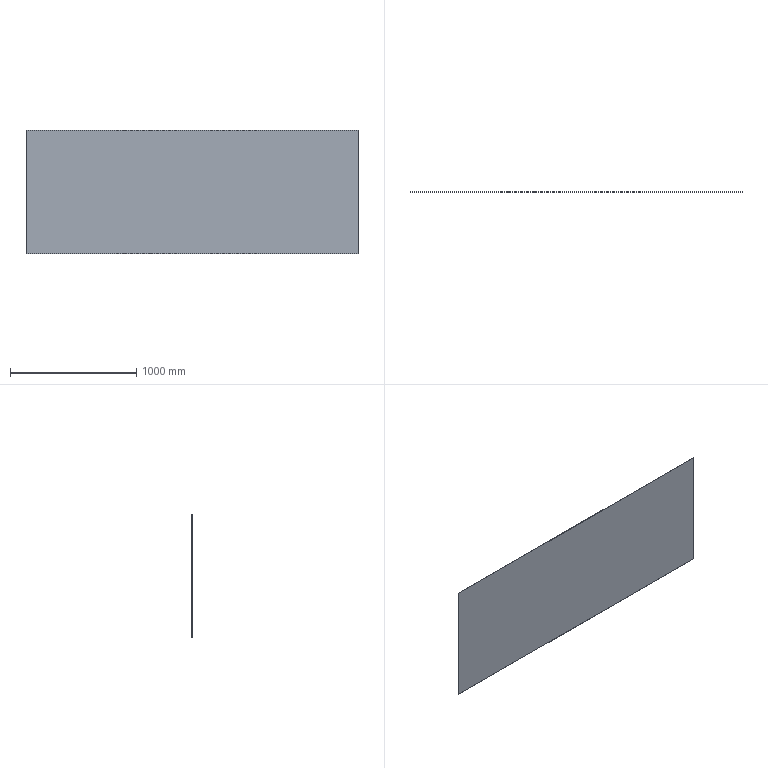Component | NX | TOP_COVER | 1 solid | 6 faces | box 2630 x 2 x 980 mm | volume 5154800 mm3 | plane 6
STEP:
#1=CARTESIAN_POINT('',(0.,0.,0.));
#2=DIRECTION('',(0.,0.,1.));
#3=DIRECTION('',(1.,0.,0.));
#4=AXIS2_PLACEMENT_3D('',#1,#2,#3);
#5=CARTESIAN_POINT('',(1972.985,1609.529,-1766.475));
#6=VERTEX_POINT('',#5);
#7=CARTESIAN_POINT('',(-657.015,1609.529,-1766.475));
#8=VERTEX_POINT('',#7);
#9=CARTESIAN_POINT('',(1972.985,1609.529,-1766.475));
#10=DIRECTION('',(-1.,0.,-0.));
#11=VECTOR('',#10,1.);
#12=LINE('',#9,#11);
#13=CARTESIAN_POINT('',(1972.985,1611.529,-1766.475));
#14=DIRECTION('',(-0.,0.,1.));
#15=DIRECTION('',(-1.,0.,-0.));
#16=AXIS2_PLACEMENT_3D('',#13,#14,#15);
#17=PLANE('',#16);
#18=CARTESIAN_POINT('',(0.,2.));
#19=DIRECTION('',(1.,0.));
#20=VECTOR('',#19,1.);
#21=LINE('',#18,#20);
#22=(GEOMETRIC_REPRESENTATION_CONTEXT(2)PARAMETRIC_REPRESENTATION_CONTEXT()REPRESENTATION_CONTEXT('',''));
#23=DEFINITIONAL_REPRESENTATION('',(#21),#22);
#24=PCURVE('',#17,#23);
#25=CARTESIAN_POINT('',(-657.015,1609.529,-2746.475));
#26=DIRECTION('',(0.,-1.,0.));
#27=DIRECTION('',(1.,0.,0.));
#28=AXIS2_PLACEMENT_3D('',#25,#26,#27);
#29=PLANE('',#28);
#30=CARTESIAN_POINT('',(2630.,980.));
#31=DIRECTION('',(-1.,-0.));
#32=VECTOR('',#31,1.);
#33=LINE('',#30,#32);
#34=(GEOMETRIC_REPRESENTATION_CONTEXT(2)PARAMETRIC_REPRESENTATION_CONTEXT()REPRESENTATION_CONTEXT('',''));
#35=DEFINITIONAL_REPRESENTATION('',(#33),#34);
#36=PCURVE('',#29,#35);
#37=SURFACE_CURVE('',#12,(#24,#36),.PCURVE_S1.);
#38=EDGE_CURVE('',#6,#8,#37,.T.);
#39=ORIENTED_EDGE('',*,*,#38,.F.);
#40=CARTESIAN_POINT('',(1972.985,1611.529,-1766.475));
#41=VERTEX_POINT('',#40);
#42=CARTESIAN_POINT('',(1972.985,1611.529,-1766.475));
#43=DIRECTION('',(0.,-1.,0.));
#44=VECTOR('',#43,1.);
#45=LINE('',#42,#44);
#46=CARTESIAN_POINT('',(0.,0.));
#47=DIRECTION('',(0.,1.));
#48=VECTOR('',#47,1.);
#49=LINE('',#46,#48);
#50=(GEOMETRIC_REPRESENTATION_CONTEXT(2)PARAMETRIC_REPRESENTATION_CONTEXT()REPRESENTATION_CONTEXT('',''));
#51=DEFINITIONAL_REPRESENTATION('',(#49),#50);
#52=PCURVE('',#17,#51);
#53=CARTESIAN_POINT('',(1972.985,1611.529,-2746.475));
#54=DIRECTION('',(1.,0.,0.));
#55=DIRECTION('',(0.,1.,0.));
#56=AXIS2_PLACEMENT_3D('',#53,#54,#55);
#57=PLANE('',#56);
#58=CARTESIAN_POINT('',(0.,980.));
#59=DIRECTION('',(-1.,0.));
#60=VECTOR('',#59,1.);
#61=LINE('',#58,#60);
#62=(GEOMETRIC_REPRESENTATION_CONTEXT(2)PARAMETRIC_REPRESENTATION_CONTEXT()REPRESENTATION_CONTEXT('',''));
#63=DEFINITIONAL_REPRESENTATION('',(#61),#62);
#64=PCURVE('',#57,#63);
#65=SURFACE_CURVE('',#45,(#52,#64),.PCURVE_S1.);
#66=EDGE_CURVE('',#41,#6,#65,.T.);
#67=ORIENTED_EDGE('',*,*,#66,.F.);
#68=CARTESIAN_POINT('',(-657.015,1611.529,-1766.475));
#69=VERTEX_POINT('',#68);
#70=CARTESIAN_POINT('',(1972.985,1611.529,-1766.475));
#71=DIRECTION('',(-1.,0.,-0.));
#72=VECTOR('',#71,1.);
#73=LINE('',#70,#72);
#74=CARTESIAN_POINT('',(0.,0.));
#75=DIRECTION('',(1.,0.));
#76=VECTOR('',#75,1.);
#77=LINE('',#74,#76);
#78=(GEOMETRIC_REPRESENTATION_CONTEXT(2)PARAMETRIC_REPRESENTATION_CONTEXT()REPRESENTATION_CONTEXT('',''));
#79=DEFINITIONAL_REPRESENTATION('',(#77),#78);
#80=PCURVE('',#17,#79);
#81=CARTESIAN_POINT('',(-657.015,1611.529,-2746.475));
#82=DIRECTION('',(0.,-1.,0.));
#83=DIRECTION('',(1.,0.,0.));
#84=AXIS2_PLACEMENT_3D('',#81,#82,#83);
#85=PLANE('',#84);
#86=CARTESIAN_POINT('',(2630.,980.));
#87=DIRECTION('',(-1.,-0.));
#88=VECTOR('',#87,1.);
#89=LINE('',#86,#88);
#90=(GEOMETRIC_REPRESENTATION_CONTEXT(2)PARAMETRIC_REPRESENTATION_CONTEXT()REPRESENTATION_CONTEXT('',''));
#91=DEFINITIONAL_REPRESENTATION('',(#89),#90);
#92=PCURVE('',#85,#91);
#93=SURFACE_CURVE('',#73,(#80,#92),.PCURVE_S1.);
#94=EDGE_CURVE('',#41,#69,#93,.T.);
#95=ORIENTED_EDGE('',*,*,#94,.T.);
#96=CARTESIAN_POINT('',(-657.015,1611.529,-1766.475));
#97=DIRECTION('',(0.,-1.,0.));
#98=VECTOR('',#97,1.);
#99=LINE('',#96,#98);
#100=CARTESIAN_POINT('',(2630.,0.));
#101=DIRECTION('',(0.,1.));
#102=VECTOR('',#101,1.);
#103=LINE('',#100,#102);
#104=(GEOMETRIC_REPRESENTATION_CONTEXT(2)PARAMETRIC_REPRESENTATION_CONTEXT()REPRESENTATION_CONTEXT('',''));
#105=DEFINITIONAL_REPRESENTATION('',(#103),#104);
#106=PCURVE('',#17,#105);
#107=CARTESIAN_POINT('',(-657.015,1611.529,-1766.475));
#108=DIRECTION('',(-1.,0.,0.));
#109=DIRECTION('',(0.,-1.,0.));
#110=AXIS2_PLACEMENT_3D('',#107,#108,#109);
#111=PLANE('',#110);
#112=CARTESIAN_POINT('',(0.,0.));
#113=DIRECTION('',(1.,0.));
#114=VECTOR('',#113,1.);
#115=LINE('',#112,#114);
#116=(GEOMETRIC_REPRESENTATION_CONTEXT(2)PARAMETRIC_REPRESENTATION_CONTEXT()REPRESENTATION_CONTEXT('',''));
#117=DEFINITIONAL_REPRESENTATION('',(#115),#116);
#118=PCURVE('',#111,#117);
#119=SURFACE_CURVE('',#99,(#106,#118),.PCURVE_S1.);
#120=EDGE_CURVE('',#69,#8,#119,.T.);
#121=ORIENTED_EDGE('',*,*,#120,.T.);
#122=EDGE_LOOP('',(#39,#67,#95,#121));
#123=FACE_BOUND('',#122,.T.);
#124=ADVANCED_FACE('',(#123),#17,.T.);
#125=CARTESIAN_POINT('',(-657.015,1609.529,-2746.475));
#126=VERTEX_POINT('',#125);
#127=CARTESIAN_POINT('',(-657.015,1609.529,-1766.475));
#128=DIRECTION('',(0.,0.,-1.));
#129=VECTOR('',#128,1.);
#130=LINE('',#127,#129);
#131=CARTESIAN_POINT('',(2.,0.));
#132=DIRECTION('',(0.,-1.));
#133=VECTOR('',#132,1.);
#134=LINE('',#131,#133);
#135=(GEOMETRIC_REPRESENTATION_CONTEXT(2)PARAMETRIC_REPRESENTATION_CONTEXT()REPRESENTATION_CONTEXT('',''));
#136=DEFINITIONAL_REPRESENTATION('',(#134),#135);
#137=PCURVE('',#111,#136);
#138=CARTESIAN_POINT('',(0.,980.));
#139=DIRECTION('',(0.,-1.));
#140=VECTOR('',#139,1.);
#141=LINE('',#138,#140);
#142=(GEOMETRIC_REPRESENTATION_CONTEXT(2)PARAMETRIC_REPRESENTATION_CONTEXT()REPRESENTATION_CONTEXT('',''));
#143=DEFINITIONAL_REPRESENTATION('',(#141),#142);
#144=PCURVE('',#29,#143);
#145=SURFACE_CURVE('',#130,(#137,#144),.PCURVE_S1.);
#146=EDGE_CURVE('',#8,#126,#145,.T.);
#147=ORIENTED_EDGE('',*,*,#146,.F.);
#148=ORIENTED_EDGE('',*,*,#120,.F.);
#149=CARTESIAN_POINT('',(-657.015,1611.529,-2746.475));
#150=VERTEX_POINT('',#149);
#151=CARTESIAN_POINT('',(-657.015,1611.529,-1766.475));
#152=DIRECTION('',(0.,0.,-1.));
#153=VECTOR('',#152,1.);
#154=LINE('',#151,#153);
#155=CARTESIAN_POINT('',(0.,0.));
#156=DIRECTION('',(0.,-1.));
#157=VECTOR('',#156,1.);
#158=LINE('',#155,#157);
#159=(GEOMETRIC_REPRESENTATION_CONTEXT(2)PARAMETRIC_REPRESENTATION_CONTEXT()REPRESENTATION_CONTEXT('',''));
#160=DEFINITIONAL_REPRESENTATION('',(#158),#159);
#161=PCURVE('',#111,#160);
#162=CARTESIAN_POINT('',(0.,980.));
#163=DIRECTION('',(0.,-1.));
#164=VECTOR('',#163,1.);
#165=LINE('',#162,#164);
#166=(GEOMETRIC_REPRESENTATION_CONTEXT(2)PARAMETRIC_REPRESENTATION_CONTEXT()REPRESENTATION_CONTEXT('',''));
#167=DEFINITIONAL_REPRESENTATION('',(#165),#166);
#168=PCURVE('',#85,#167);
#169=SURFACE_CURVE('',#154,(#161,#168),.PCURVE_S1.);
#170=EDGE_CURVE('',#69,#150,#169,.T.);
#171=ORIENTED_EDGE('',*,*,#170,.T.);
#172=CARTESIAN_POINT('',(-657.015,1611.529,-2746.475));
#173=DIRECTION('',(0.,-1.,0.));
#174=VECTOR('',#173,1.);
#175=LINE('',#172,#174);
#176=CARTESIAN_POINT('',(0.,-980.));
#177=DIRECTION('',(1.,0.));
#178=VECTOR('',#177,1.);
#179=LINE('',#176,#178);
#180=(GEOMETRIC_REPRESENTATION_CONTEXT(2)PARAMETRIC_REPRESENTATION_CONTEXT()REPRESENTATION_CONTEXT('',''));
#181=DEFINITIONAL_REPRESENTATION('',(#179),#180);
#182=PCURVE('',#111,#181);
#183=CARTESIAN_POINT('',(-657.015,1611.529,-2746.475));
#184=DIRECTION('',(0.,0.,-1.));
#185=DIRECTION('',(1.,0.,0.));
#186=AXIS2_PLACEMENT_3D('',#183,#184,#185);
#187=PLANE('',#186);
#188=CARTESIAN_POINT('',(0.,0.));
#189=DIRECTION('',(0.,1.));
#190=VECTOR('',#189,1.);
#191=LINE('',#188,#190);
#192=(GEOMETRIC_REPRESENTATION_CONTEXT(2)PARAMETRIC_REPRESENTATION_CONTEXT()REPRESENTATION_CONTEXT('',''));
#193=DEFINITIONAL_REPRESENTATION('',(#191),#192);
#194=PCURVE('',#187,#193);
#195=SURFACE_CURVE('',#175,(#182,#194),.PCURVE_S1.);
#196=EDGE_CURVE('',#150,#126,#195,.T.);
#197=ORIENTED_EDGE('',*,*,#196,.T.);
#198=EDGE_LOOP('',(#147,#148,#171,#197));
#199=FACE_BOUND('',#198,.T.);
#200=ADVANCED_FACE('',(#199),#111,.T.);
#201=CARTESIAN_POINT('',(1972.985,1609.529,-2746.475));
#202=VERTEX_POINT('',#201);
#203=CARTESIAN_POINT('',(-657.015,1609.529,-2746.475));
#204=DIRECTION('',(1.,0.,0.));
#205=VECTOR('',#204,1.);
#206=LINE('',#203,#205);
#207=CARTESIAN_POINT('',(0.,2.));
#208=DIRECTION('',(1.,0.));
#209=VECTOR('',#208,1.);
#210=LINE('',#207,#209);
#211=(GEOMETRIC_REPRESENTATION_CONTEXT(2)PARAMETRIC_REPRESENTATION_CONTEXT()REPRESENTATION_CONTEXT('',''));
#212=DEFINITIONAL_REPRESENTATION('',(#210),#211);
#213=PCURVE('',#187,#212);
#214=CARTESIAN_POINT('',(0.,0.));
#215=DIRECTION('',(1.,0.));
#216=VECTOR('',#215,1.);
#217=LINE('',#214,#216);
#218=(GEOMETRIC_REPRESENTATION_CONTEXT(2)PARAMETRIC_REPRESENTATION_CONTEXT()REPRESENTATION_CONTEXT('',''));
#219=DEFINITIONAL_REPRESENTATION('',(#217),#218);
#220=PCURVE('',#29,#219);
#221=SURFACE_CURVE('',#206,(#213,#220),.PCURVE_S1.);
#222=EDGE_CURVE('',#126,#202,#221,.T.);
#223=ORIENTED_EDGE('',*,*,#222,.F.);
#224=ORIENTED_EDGE('',*,*,#196,.F.);
#225=CARTESIAN_POINT('',(1972.985,1611.529,-2746.475));
#226=VERTEX_POINT('',#225);
#227=CARTESIAN_POINT('',(-657.015,1611.529,-2746.475));
#228=DIRECTION('',(1.,0.,0.));
#229=VECTOR('',#228,1.);
#230=LINE('',#227,#229);
#231=CARTESIAN_POINT('',(0.,0.));
#232=DIRECTION('',(1.,0.));
#233=VECTOR('',#232,1.);
#234=LINE('',#231,#233);
#235=(GEOMETRIC_REPRESENTATION_CONTEXT(2)PARAMETRIC_REPRESENTATION_CONTEXT()REPRESENTATION_CONTEXT('',''));
#236=DEFINITIONAL_REPRESENTATION('',(#234),#235);
#237=PCURVE('',#187,#236);
#238=CARTESIAN_POINT('',(0.,0.));
#239=DIRECTION('',(1.,0.));
#240=VECTOR('',#239,1.);
#241=LINE('',#238,#240);
#242=(GEOMETRIC_REPRESENTATION_CONTEXT(2)PARAMETRIC_REPRESENTATION_CONTEXT()REPRESENTATION_CONTEXT('',''));
#243=DEFINITIONAL_REPRESENTATION('',(#241),#242);
#244=PCURVE('',#85,#243);
#245=SURFACE_CURVE('',#230,(#237,#244),.PCURVE_S1.);
#246=EDGE_CURVE('',#150,#226,#245,.T.);
#247=ORIENTED_EDGE('',*,*,#246,.T.);
#248=CARTESIAN_POINT('',(1972.985,1611.529,-2746.475));
#249=DIRECTION('',(0.,-1.,0.));
#250=VECTOR('',#249,1.);
#251=LINE('',#248,#250);
#252=CARTESIAN_POINT('',(2630.,0.));
#253=DIRECTION('',(0.,1.));
#254=VECTOR('',#253,1.);
#255=LINE('',#252,#254);
#256=(GEOMETRIC_REPRESENTATION_CONTEXT(2)PARAMETRIC_REPRESENTATION_CONTEXT()REPRESENTATION_CONTEXT('',''));
#257=DEFINITIONAL_REPRESENTATION('',(#255),#256);
#258=PCURVE('',#187,#257);
#259=CARTESIAN_POINT('',(0.,0.));
#260=DIRECTION('',(-1.,0.));
#261=VECTOR('',#260,1.);
#262=LINE('',#259,#261);
#263=(GEOMETRIC_REPRESENTATION_CONTEXT(2)PARAMETRIC_REPRESENTATION_CONTEXT()REPRESENTATION_CONTEXT('',''));
#264=DEFINITIONAL_REPRESENTATION('',(#262),#263);
#265=PCURVE('',#57,#264);
#266=SURFACE_CURVE('',#251,(#258,#265),.PCURVE_S1.);
#267=EDGE_CURVE('',#226,#202,#266,.T.);
#268=ORIENTED_EDGE('',*,*,#267,.T.);
#269=EDGE_LOOP('',(#223,#224,#247,#268));
#270=FACE_BOUND('',#269,.T.);
#271=ADVANCED_FACE('',(#270),#187,.T.);
#272=CARTESIAN_POINT('',(1972.985,1609.529,-2746.475));
#273=DIRECTION('',(0.,0.,1.));
#274=VECTOR('',#273,1.);
#275=LINE('',#272,#274);
#276=CARTESIAN_POINT('',(-2.,0.));
#277=DIRECTION('',(0.,1.));
#278=VECTOR('',#277,1.);
#279=LINE('',#276,#278);
#280=(GEOMETRIC_REPRESENTATION_CONTEXT(2)PARAMETRIC_REPRESENTATION_CONTEXT()REPRESENTATION_CONTEXT('',''));
#281=DEFINITIONAL_REPRESENTATION('',(#279),#280);
#282=PCURVE('',#57,#281);
#283=CARTESIAN_POINT('',(2630.,0.));
#284=DIRECTION('',(0.,1.));
#285=VECTOR('',#284,1.);
#286=LINE('',#283,#285);
#287=(GEOMETRIC_REPRESENTATION_CONTEXT(2)PARAMETRIC_REPRESENTATION_CONTEXT()REPRESENTATION_CONTEXT('',''));
#288=DEFINITIONAL_REPRESENTATION('',(#286),#287);
#289=PCURVE('',#29,#288);
#290=SURFACE_CURVE('',#275,(#282,#289),.PCURVE_S1.);
#291=EDGE_CURVE('',#202,#6,#290,.T.);
#292=ORIENTED_EDGE('',*,*,#291,.F.);
#293=ORIENTED_EDGE('',*,*,#267,.F.);
#294=CARTESIAN_POINT('',(1972.985,1611.529,-2746.475));
#295=DIRECTION('',(0.,0.,1.));
#296=VECTOR('',#295,1.);
#297=LINE('',#294,#296);
#298=CARTESIAN_POINT('',(0.,0.));
#299=DIRECTION('',(0.,1.));
#300=VECTOR('',#299,1.);
#301=LINE('',#298,#300);
#302=(GEOMETRIC_REPRESENTATION_CONTEXT(2)PARAMETRIC_REPRESENTATION_CONTEXT()REPRESENTATION_CONTEXT('',''));
#303=DEFINITIONAL_REPRESENTATION('',(#301),#302);
#304=PCURVE('',#57,#303);
#305=CARTESIAN_POINT('',(2630.,0.));
#306=DIRECTION('',(0.,1.));
#307=VECTOR('',#306,1.);
#308=LINE('',#305,#307);
#309=(GEOMETRIC_REPRESENTATION_CONTEXT(2)PARAMETRIC_REPRESENTATION_CONTEXT()REPRESENTATION_CONTEXT('',''));
#310=DEFINITIONAL_REPRESENTATION('',(#308),#309);
#311=PCURVE('',#85,#310);
#312=SURFACE_CURVE('',#297,(#304,#311),.PCURVE_S1.);
#313=EDGE_CURVE('',#226,#41,#312,.T.);
#314=ORIENTED_EDGE('',*,*,#313,.T.);
#315=ORIENTED_EDGE('',*,*,#66,.T.);
#316=EDGE_LOOP('',(#292,#293,#314,#315));
#317=FACE_BOUND('',#316,.T.);
#318=ADVANCED_FACE('',(#317),#57,.T.);
#319=ORIENTED_EDGE('',*,*,#94,.F.);
#320=ORIENTED_EDGE('',*,*,#313,.F.);
#321=ORIENTED_EDGE('',*,*,#246,.F.);
#322=ORIENTED_EDGE('',*,*,#170,.F.);
#323=EDGE_LOOP('',(#319,#320,#321,#322));
#324=FACE_BOUND('',#323,.T.);
#325=ADVANCED_FACE('',(#324),#85,.F.);
#326=ORIENTED_EDGE('',*,*,#38,.T.);
#327=ORIENTED_EDGE('',*,*,#146,.T.);
#328=ORIENTED_EDGE('',*,*,#222,.T.);
#329=ORIENTED_EDGE('',*,*,#291,.T.);
#330=EDGE_LOOP('',(#326,#327,#328,#329));
#331=FACE_BOUND('',#330,.T.);
#332=ADVANCED_FACE('',(#331),#29,.T.);
#333=CLOSED_SHELL('',(#124,#200,#271,#318,#325,#332));
#334=MANIFOLD_SOLID_BREP('',#333);
#335=(LENGTH_UNIT()NAMED_UNIT(*)SI_UNIT(.MILLI.,.METRE.));
#336=UNCERTAINTY_MEASURE_WITH_UNIT(LENGTH_MEASURE(0.0000001),#335,'','');
#337=(NAMED_UNIT(*)PLANE_ANGLE_UNIT()SI_UNIT($,.RADIAN.));
#338=(NAMED_UNIT(*)SI_UNIT($,.STERADIAN.)SOLID_ANGLE_UNIT());
#339=(GEOMETRIC_REPRESENTATION_CONTEXT(3)GLOBAL_UNCERTAINTY_ASSIGNED_CONTEXT((#336))GLOBAL_UNIT_ASSIGNED_CONTEXT((#335,#337,#338))REPRESENTATION_CONTEXT('',''));
#340=ADVANCED_BREP_SHAPE_REPRESENTATION('',(#4,#334),#339);